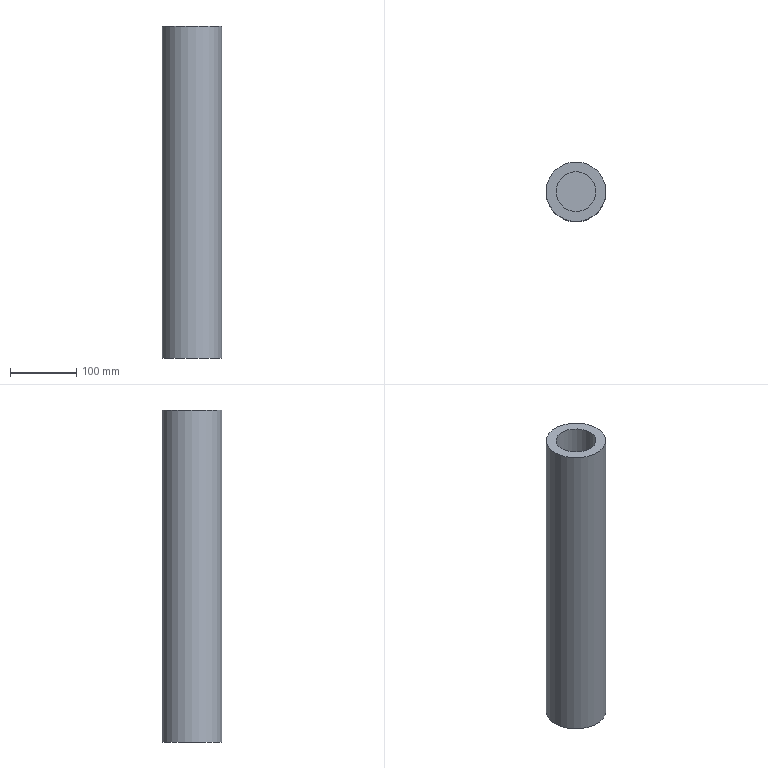Component | NX | LOWER_LINK_ROD | 1 solid | 5 faces | box 90 x 90 x 500 mm | volume 3039491 mm3 | plane 3 | cylinder 2 | commonest cylinder face diameters 90 x1 60 x1
STEP:
#1=CARTESIAN_POINT('',(0.,0.,0.));
#2=DIRECTION('',(0.,0.,1.));
#3=DIRECTION('',(1.,0.,0.));
#4=AXIS2_PLACEMENT_3D('',#1,#2,#3);
#5=CARTESIAN_POINT('',(-45.,-0.,-622.5));
#6=VERTEX_POINT('',#5);
#7=CARTESIAN_POINT('',(0.,-0.,-622.5));
#8=DIRECTION('',(0.,0.,-1.));
#9=DIRECTION('',(-1.,-0.,0.));
#10=AXIS2_PLACEMENT_3D('',#7,#8,#9);
#11=CIRCLE('',#10,45.);
#12=CARTESIAN_POINT('',(0.,-0.,-622.5));
#13=DIRECTION('',(0.,0.,-1.));
#14=DIRECTION('',(1.,0.,0.));
#15=AXIS2_PLACEMENT_3D('',#12,#13,#14);
#16=CYLINDRICAL_SURFACE('',#15,45.);
#17=CARTESIAN_POINT('',(3.142,0.));
#18=DIRECTION('',(1.,0.));
#19=VECTOR('',#18,1.);
#20=LINE('',#17,#19);
#21=(GEOMETRIC_REPRESENTATION_CONTEXT(2)PARAMETRIC_REPRESENTATION_CONTEXT()REPRESENTATION_CONTEXT('',''));
#22=DEFINITIONAL_REPRESENTATION('',(#20),#21);
#23=PCURVE('',#16,#22);
#24=CARTESIAN_POINT('',(0.,-0.,-622.5));
#25=DIRECTION('',(0.,0.,-1.));
#26=DIRECTION('',(1.,0.,0.));
#27=AXIS2_PLACEMENT_3D('',#24,#25,#26);
#28=PLANE('',#27);
#29=CARTESIAN_POINT('',(0.,0.));
#30=DIRECTION('',(-1.,0.));
#31=AXIS2_PLACEMENT_2D('',#29,#30);
#32=CIRCLE('',#31,45.);
#33=(GEOMETRIC_REPRESENTATION_CONTEXT(2)PARAMETRIC_REPRESENTATION_CONTEXT()REPRESENTATION_CONTEXT('',''));
#34=DEFINITIONAL_REPRESENTATION('',(#32),#33);
#35=PCURVE('',#28,#34);
#36=SURFACE_CURVE('',#11,(#23,#35),.PCURVE_S1.);
#37=EDGE_CURVE('',#6,#6,#36,.T.);
#38=ORIENTED_EDGE('',*,*,#37,.T.);
#39=CARTESIAN_POINT('',(-45.,-0.,-1122.5));
#40=VERTEX_POINT('',#39);
#41=CARTESIAN_POINT('',(-45.,-0.,-622.5));
#42=CARTESIAN_POINT('',(-45.,-0.,-1122.5));
#43=B_SPLINE_CURVE_WITH_KNOTS('',1,(#41,#42),.UNSPECIFIED.,.F.,.F.,(2,2),(0.,500.),.PIECEWISE_BEZIER_KNOTS.);
#44=CARTESIAN_POINT('',(9.425,0.));
#45=DIRECTION('',(0.,1.));
#46=VECTOR('',#45,1.);
#47=LINE('',#44,#46);
#48=(GEOMETRIC_REPRESENTATION_CONTEXT(2)PARAMETRIC_REPRESENTATION_CONTEXT()REPRESENTATION_CONTEXT('',''));
#49=DEFINITIONAL_REPRESENTATION('',(#47),#48);
#50=PCURVE('',#16,#49);
#51=CARTESIAN_POINT('',(3.142,0.));
#52=DIRECTION('',(0.,1.));
#53=VECTOR('',#52,1.);
#54=LINE('',#51,#53);
#55=(GEOMETRIC_REPRESENTATION_CONTEXT(2)PARAMETRIC_REPRESENTATION_CONTEXT()REPRESENTATION_CONTEXT('',''));
#56=DEFINITIONAL_REPRESENTATION('',(#54),#55);
#57=PCURVE('',#16,#56);
#58=SEAM_CURVE('',#43,(#50,#57),.PCURVE_S1.);
#59=EDGE_CURVE('',#6,#40,#58,.T.);
#60=ORIENTED_EDGE('',*,*,#59,.T.);
#61=CARTESIAN_POINT('',(0.,-0.,-1122.5));
#62=DIRECTION('',(0.,0.,-1.));
#63=DIRECTION('',(-1.,-0.,0.));
#64=AXIS2_PLACEMENT_3D('',#61,#62,#63);
#65=CIRCLE('',#64,45.);
#66=CARTESIAN_POINT('',(3.142,500.));
#67=DIRECTION('',(1.,0.));
#68=VECTOR('',#67,1.);
#69=LINE('',#66,#68);
#70=(GEOMETRIC_REPRESENTATION_CONTEXT(2)PARAMETRIC_REPRESENTATION_CONTEXT()REPRESENTATION_CONTEXT('',''));
#71=DEFINITIONAL_REPRESENTATION('',(#69),#70);
#72=PCURVE('',#16,#71);
#73=CARTESIAN_POINT('',(0.,-0.,-1122.5));
#74=DIRECTION('',(0.,0.,-1.));
#75=DIRECTION('',(1.,0.,0.));
#76=AXIS2_PLACEMENT_3D('',#73,#74,#75);
#77=PLANE('',#76);
#78=CARTESIAN_POINT('',(0.,0.));
#79=DIRECTION('',(-1.,0.));
#80=AXIS2_PLACEMENT_2D('',#78,#79);
#81=CIRCLE('',#80,45.);
#82=(GEOMETRIC_REPRESENTATION_CONTEXT(2)PARAMETRIC_REPRESENTATION_CONTEXT()REPRESENTATION_CONTEXT('',''));
#83=DEFINITIONAL_REPRESENTATION('',(#81),#82);
#84=PCURVE('',#77,#83);
#85=SURFACE_CURVE('',#65,(#72,#84),.PCURVE_S1.);
#86=EDGE_CURVE('',#40,#40,#85,.T.);
#87=ORIENTED_EDGE('',*,*,#86,.F.);
#88=ORIENTED_EDGE('',*,*,#59,.F.);
#89=EDGE_LOOP('',(#38,#60,#87,#88));
#90=FACE_BOUND('',#89,.T.);
#91=ADVANCED_FACE('',(#90),#16,.T.);
#92=CARTESIAN_POINT('',(-30.,-0.,-622.5));
#93=VERTEX_POINT('',#92);
#94=CARTESIAN_POINT('',(0.,-0.,-622.5));
#95=DIRECTION('',(0.,0.,-1.));
#96=DIRECTION('',(-1.,-0.,0.));
#97=AXIS2_PLACEMENT_3D('',#94,#95,#96);
#98=CIRCLE('',#97,30.);
#99=CARTESIAN_POINT('',(0.,0.));
#100=DIRECTION('',(-1.,0.));
#101=AXIS2_PLACEMENT_2D('',#99,#100);
#102=CIRCLE('',#101,30.);
#103=(GEOMETRIC_REPRESENTATION_CONTEXT(2)PARAMETRIC_REPRESENTATION_CONTEXT()REPRESENTATION_CONTEXT('',''));
#104=DEFINITIONAL_REPRESENTATION('',(#102),#103);
#105=PCURVE('',#28,#104);
#106=CARTESIAN_POINT('',(0.,-0.,-672.5));
#107=DIRECTION('',(0.,0.,1.));
#108=DIRECTION('',(-1.,0.,0.));
#109=AXIS2_PLACEMENT_3D('',#106,#107,#108);
#110=CYLINDRICAL_SURFACE('',#109,30.);
#111=CARTESIAN_POINT('',(6.283,50.));
#112=DIRECTION('',(-1.,0.));
#113=VECTOR('',#112,1.);
#114=LINE('',#111,#113);
#115=(GEOMETRIC_REPRESENTATION_CONTEXT(2)PARAMETRIC_REPRESENTATION_CONTEXT()REPRESENTATION_CONTEXT('',''));
#116=DEFINITIONAL_REPRESENTATION('',(#114),#115);
#117=PCURVE('',#110,#116);
#118=SURFACE_CURVE('',#98,(#105,#117),.PCURVE_S1.);
#119=EDGE_CURVE('',#93,#93,#118,.T.);
#120=ORIENTED_EDGE('',*,*,#119,.T.);
#121=EDGE_LOOP('',(#120));
#122=FACE_BOUND('',#121,.T.);
#123=ORIENTED_EDGE('',*,*,#37,.F.);
#124=EDGE_LOOP('',(#123));
#125=FACE_BOUND('',#124,.T.);
#126=ADVANCED_FACE('',(#122,#125),#28,.F.);
#127=ORIENTED_EDGE('',*,*,#86,.T.);
#128=EDGE_LOOP('',(#127));
#129=FACE_BOUND('',#128,.T.);
#130=ADVANCED_FACE('',(#129),#77,.T.);
#131=CARTESIAN_POINT('',(-30.,-0.,-672.5));
#132=VERTEX_POINT('',#131);
#133=CARTESIAN_POINT('',(0.,-0.,-672.5));
#134=DIRECTION('',(0.,0.,1.));
#135=DIRECTION('',(-1.,-0.,0.));
#136=AXIS2_PLACEMENT_3D('',#133,#134,#135);
#137=CIRCLE('',#136,30.);
#138=CARTESIAN_POINT('',(0.,0.));
#139=DIRECTION('',(1.,0.));
#140=VECTOR('',#139,1.);
#141=LINE('',#138,#140);
#142=(GEOMETRIC_REPRESENTATION_CONTEXT(2)PARAMETRIC_REPRESENTATION_CONTEXT()REPRESENTATION_CONTEXT('',''));
#143=DEFINITIONAL_REPRESENTATION('',(#141),#142);
#144=PCURVE('',#110,#143);
#145=CARTESIAN_POINT('',(0.,-0.,-672.5));
#146=DIRECTION('',(0.,0.,-1.));
#147=DIRECTION('',(1.,0.,0.));
#148=AXIS2_PLACEMENT_3D('',#145,#146,#147);
#149=PLANE('',#148);
#150=CARTESIAN_POINT('',(-30.,0.));
#151=CARTESIAN_POINT('',(-30.,51.962));
#152=CARTESIAN_POINT('',(15.,25.981));
#153=CARTESIAN_POINT('',(60.,0.));
#154=CARTESIAN_POINT('',(15.,-25.981));
#155=CARTESIAN_POINT('',(-30.,-51.962));
#156=CARTESIAN_POINT('',(-30.,0.));
#157=(BOUNDED_CURVE()B_SPLINE_CURVE(2,(#150,#151,#152,#153,#154,#155,#156),.UNSPECIFIED.,.T.,.F.)B_SPLINE_CURVE_WITH_KNOTS((1,2,2,2,2,1),(-2.094,0.,2.094,4.189,6.283,8.378),.UNSPECIFIED.)CURVE()GEOMETRIC_REPRESENTATION_ITEM()RATIONAL_B_SPLINE_CURVE((1.,0.5,1.,0.5,1.,0.5,1.))REPRESENTATION_ITEM(''));
#158=(GEOMETRIC_REPRESENTATION_CONTEXT(2)PARAMETRIC_REPRESENTATION_CONTEXT()REPRESENTATION_CONTEXT('',''));
#159=DEFINITIONAL_REPRESENTATION('',(#157),#158);
#160=PCURVE('',#149,#159);
#161=SURFACE_CURVE('',#137,(#144,#160),.PCURVE_S1.);
#162=EDGE_CURVE('',#132,#132,#161,.T.);
#163=ORIENTED_EDGE('',*,*,#162,.T.);
#164=CARTESIAN_POINT('',(-30.,-0.,-672.5));
#165=CARTESIAN_POINT('',(-30.,-0.,-622.5));
#166=B_SPLINE_CURVE_WITH_KNOTS('',1,(#164,#165),.UNSPECIFIED.,.F.,.F.,(2,2),(0.,50.),.PIECEWISE_BEZIER_KNOTS.);
#167=CARTESIAN_POINT('',(6.283,0.));
#168=DIRECTION('',(0.,1.));
#169=VECTOR('',#168,1.);
#170=LINE('',#167,#169);
#171=(GEOMETRIC_REPRESENTATION_CONTEXT(2)PARAMETRIC_REPRESENTATION_CONTEXT()REPRESENTATION_CONTEXT('',''));
#172=DEFINITIONAL_REPRESENTATION('',(#170),#171);
#173=PCURVE('',#110,#172);
#174=CARTESIAN_POINT('',(0.,0.));
#175=DIRECTION('',(0.,1.));
#176=VECTOR('',#175,1.);
#177=LINE('',#174,#176);
#178=(GEOMETRIC_REPRESENTATION_CONTEXT(2)PARAMETRIC_REPRESENTATION_CONTEXT()REPRESENTATION_CONTEXT('',''));
#179=DEFINITIONAL_REPRESENTATION('',(#177),#178);
#180=PCURVE('',#110,#179);
#181=SEAM_CURVE('',#166,(#173,#180),.PCURVE_S1.);
#182=EDGE_CURVE('',#132,#93,#181,.T.);
#183=ORIENTED_EDGE('',*,*,#182,.T.);
#184=ORIENTED_EDGE('',*,*,#119,.T.);
#185=ORIENTED_EDGE('',*,*,#182,.F.);
#186=EDGE_LOOP('',(#163,#183,#184,#185));
#187=FACE_BOUND('',#186,.F.);
#188=ADVANCED_FACE('',(#187),#110,.F.);
#189=ORIENTED_EDGE('',*,*,#162,.T.);
#190=EDGE_LOOP('',(#189));
#191=FACE_BOUND('',#190,.T.);
#192=ADVANCED_FACE('',(#191),#149,.F.);
#193=CLOSED_SHELL('',(#91,#126,#130,#188,#192));
#194=MANIFOLD_SOLID_BREP('',#193);
#195=(LENGTH_UNIT()NAMED_UNIT(*)SI_UNIT(.MILLI.,.METRE.));
#196=UNCERTAINTY_MEASURE_WITH_UNIT(LENGTH_MEASURE(0.00001),#195,'','');
#197=(NAMED_UNIT(*)PLANE_ANGLE_UNIT()SI_UNIT($,.RADIAN.));
#198=(NAMED_UNIT(*)SI_UNIT($,.STERADIAN.)SOLID_ANGLE_UNIT());
#199=(GEOMETRIC_REPRESENTATION_CONTEXT(3)GLOBAL_UNCERTAINTY_ASSIGNED_CONTEXT((#196))GLOBAL_UNIT_ASSIGNED_CONTEXT((#195,#197,#198))REPRESENTATION_CONTEXT('',''));
#200=ADVANCED_BREP_SHAPE_REPRESENTATION('',(#4,#194),#199);